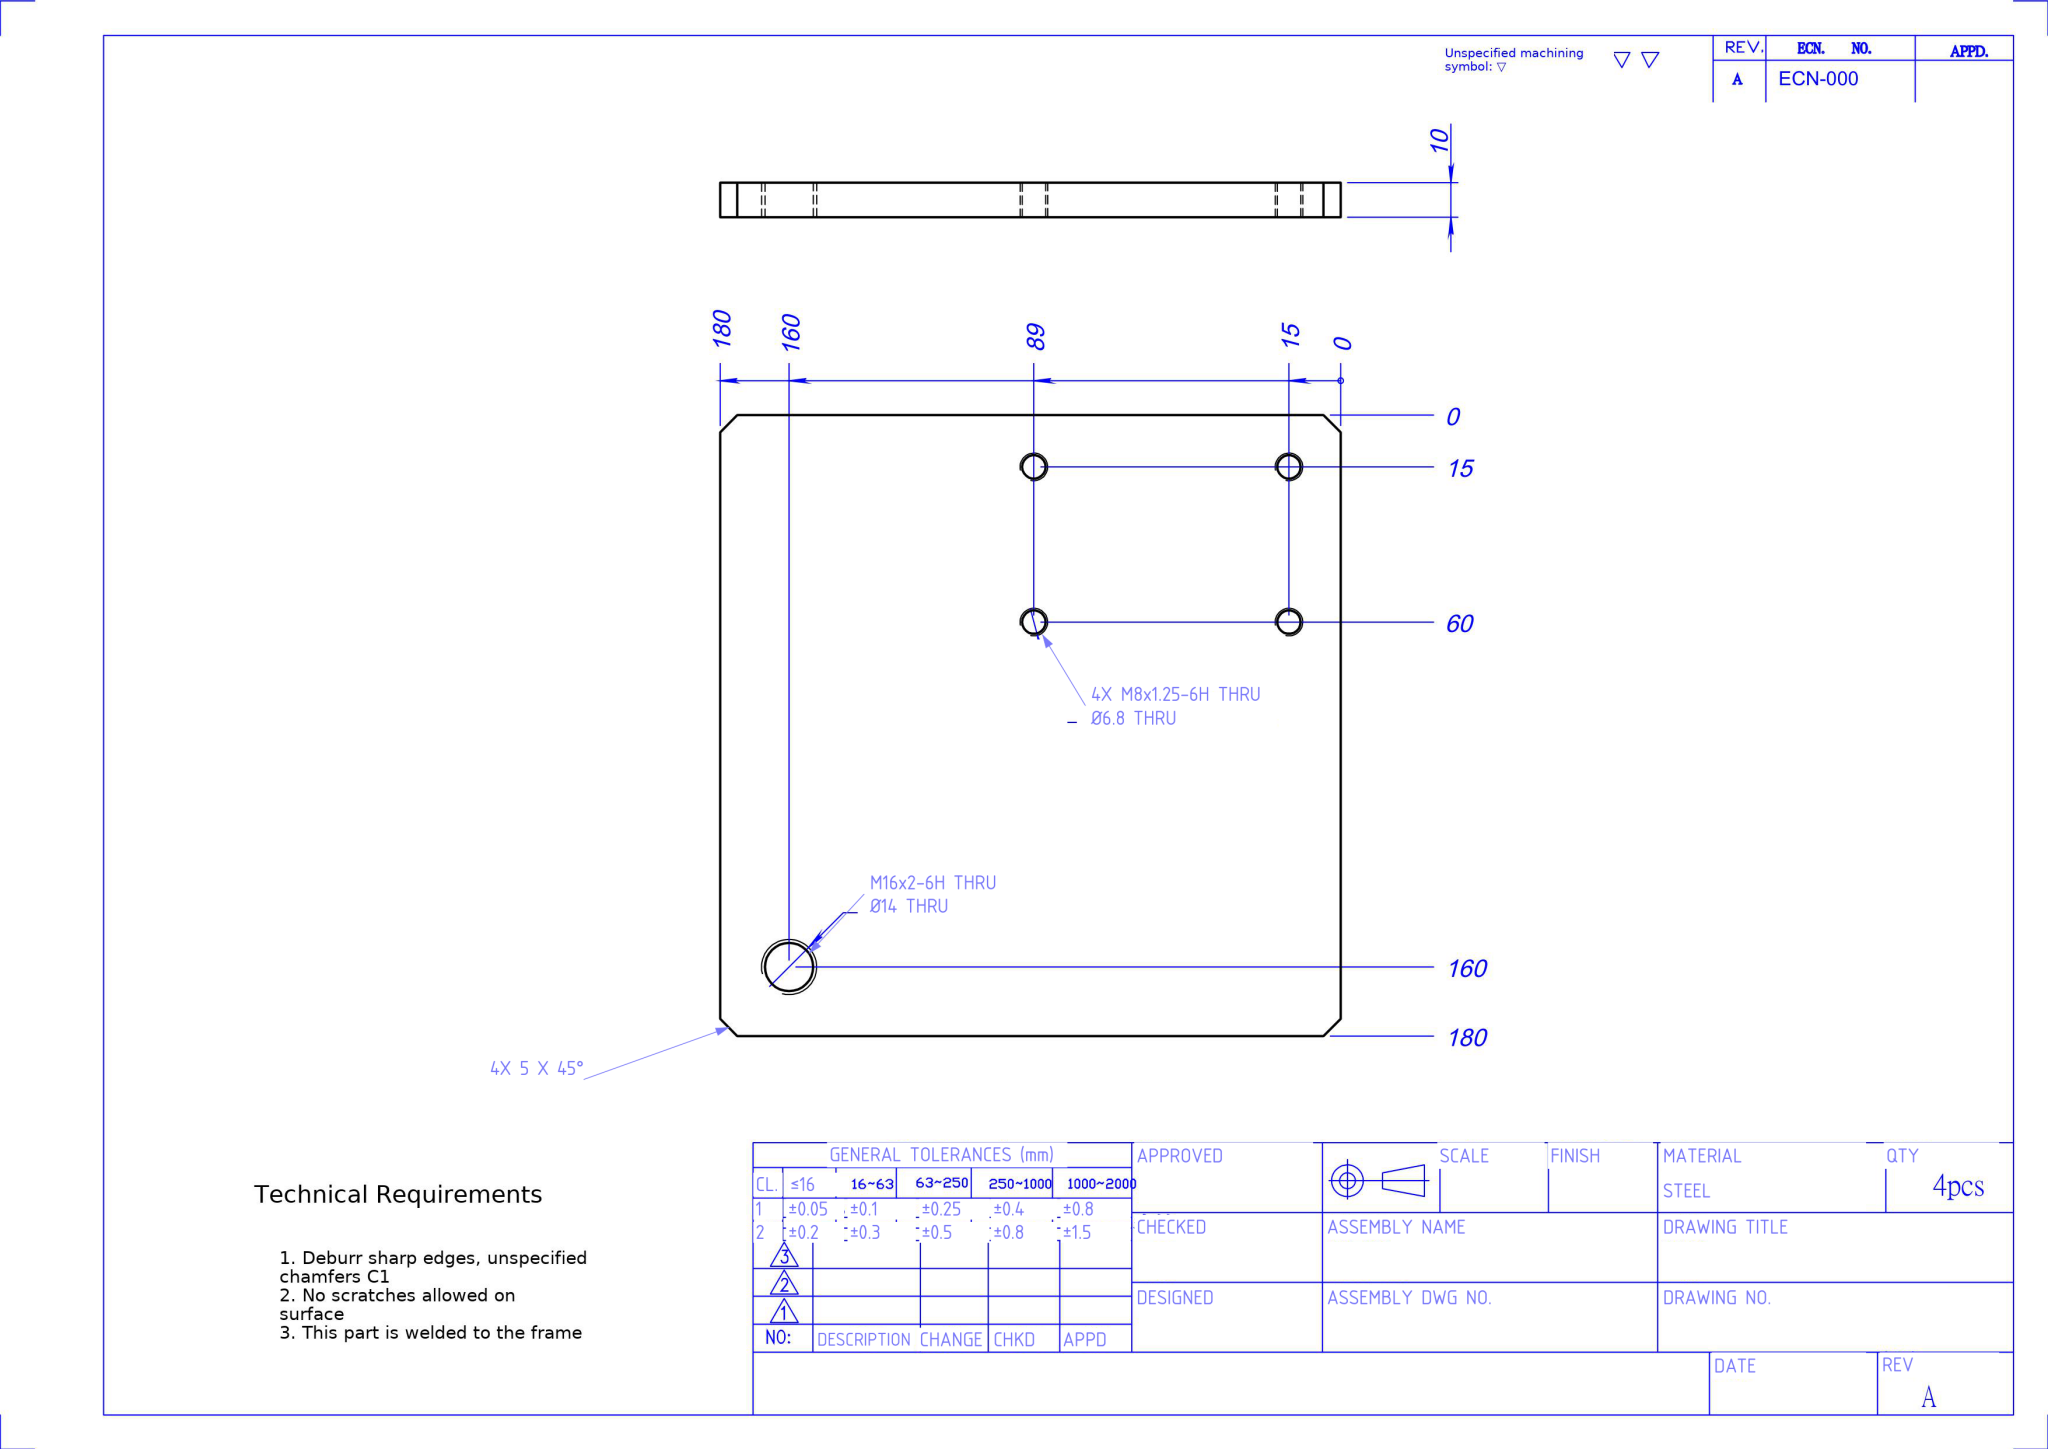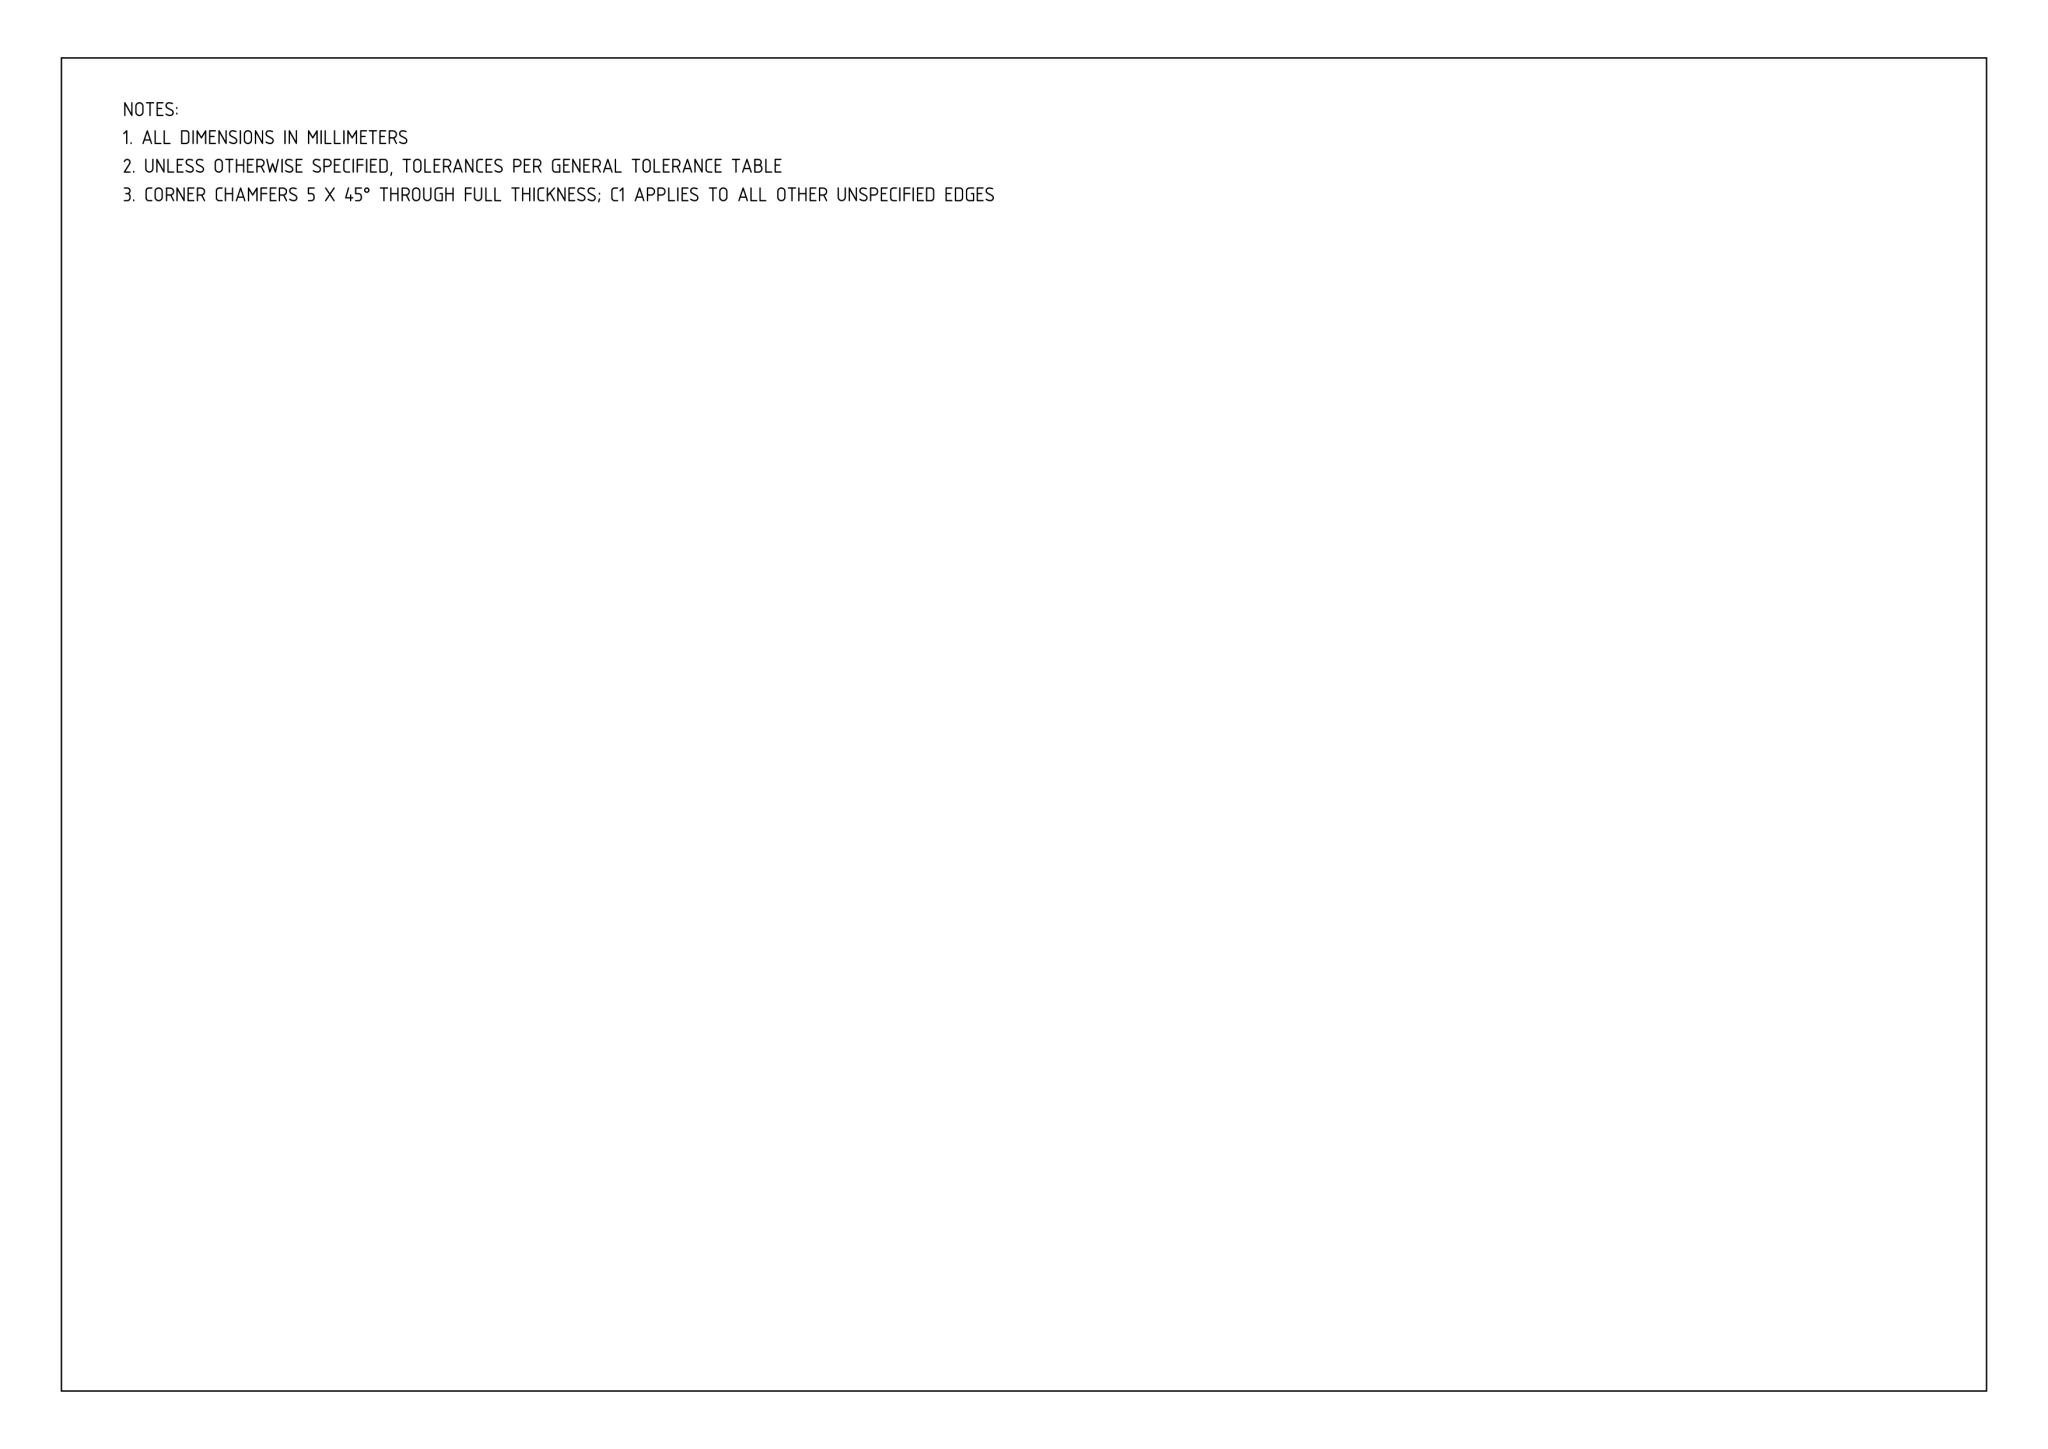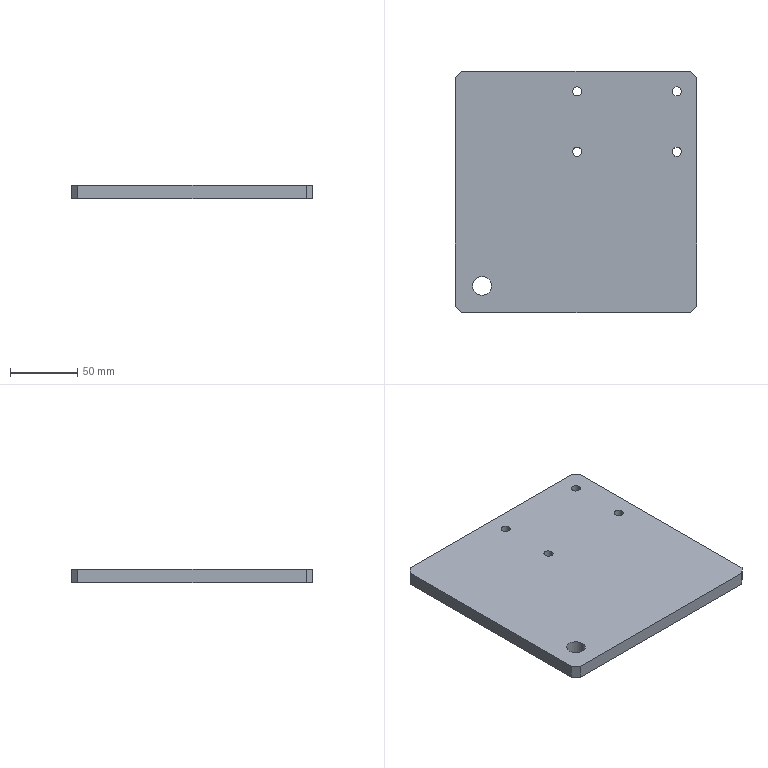Part | NX | mm | 1 solid | 20 faces | box 180 x 180 x 10 mm | volume 320508 mm3 | cylinder 10 | plane 10 | commonest cylinder face diameters 6.8 x8 14 x2